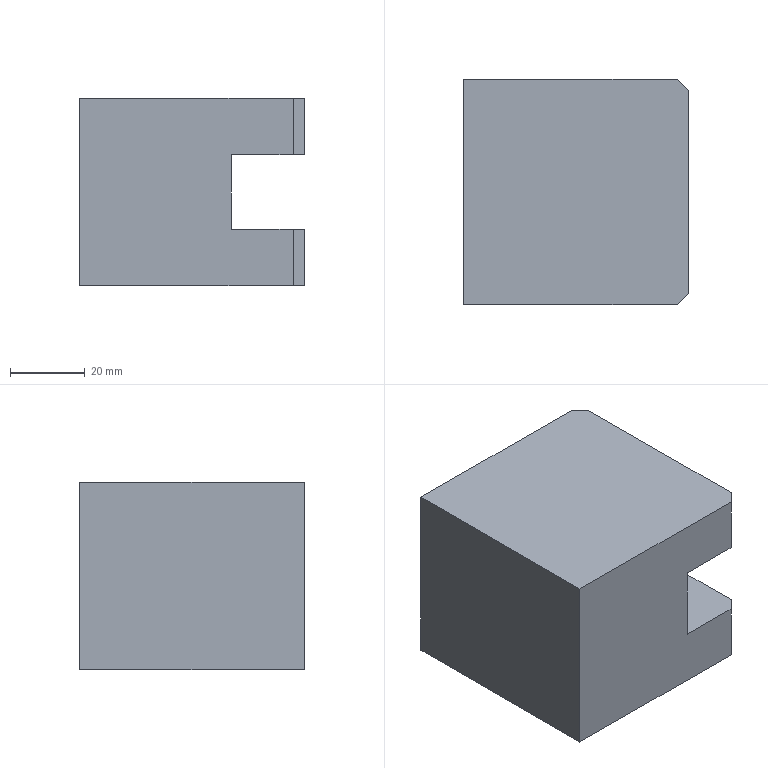Component | SolidWorks | Part52-1 | 1 solid | 14 faces | box 60 x 60 x 50 mm | volume 156330 mm3 | plane 14
build123d program:
from build123d import *

# Parameters (mm, degrees)
BOSS_EXTRUDE1_DEPTH = 30
CHAMFER1_SIZE       = 3


with BuildPart() as part:
    # Sketch1 → Boss-Extrude1 (new, symmetric)
    with BuildSketch(Plane(origin=(0, 0, 0), x_dir=(0, 0, -1), z_dir=(1, 0, 0))):
        Polygon((-25, 0), (25, 0), (25, 60), (10, 60), (10, 40.5), (-10, 40.5), (-10, 60), (-25, 60), align=None)
    extrude(amount=BOSS_EXTRUDE1_DEPTH, both=True)

    # Chamfer1
    chamfer1_edges = [part.edges().sort_by_distance(p)[0] for p in [
        (30, 60, -17.5),
        (30, 60, 17.5),
        (-30, 60, 17.5),
        (-30, 60, -17.5),
    ]]
    chamfer(chamfer1_edges, length=CHAMFER1_SIZE)


solid = part.part

# Placed as in the assembly
solid = solid.moved(Location((-265.007, 209, -385), (0, 0, -90)))
STEP:
#1=COLOUR_RGB('',0.7922,0.8196,0.9333);
#2=FILL_AREA_STYLE_COLOUR('',#1);
#3=FILL_AREA_STYLE('',(#2));
#4=SURFACE_STYLE_FILL_AREA(#3);
#5=SURFACE_SIDE_STYLE('',(#4));
#6=SURFACE_STYLE_USAGE(.BOTH.,#5);
#7=PRESENTATION_STYLE_ASSIGNMENT((#6));
#8=CARTESIAN_POINT('',(-8.071,7.165,-14.173));
#9=VERTEX_POINT('',#8);
#10=CARTESIAN_POINT('',(-8.071,9.291,-14.173));
#11=VERTEX_POINT('',#10);
#12=CARTESIAN_POINT('',(-8.071,7.047,-14.173));
#13=DIRECTION('',(0.,1.,0.));
#14=VECTOR('',#13,39.37);
#15=LINE('',#12,#14);
#16=EDGE_CURVE('',#9,#11,#15,.T.);
#17=ORIENTED_EDGE('',*,*,#16,.T.);
#18=CARTESIAN_POINT('',(-8.189,9.409,-14.173));
#19=VERTEX_POINT('',#18);
#20=CARTESIAN_POINT('',(-8.071,9.291,-14.173));
#21=DIRECTION('',(-0.7071,0.7071,0.));
#22=VECTOR('',#21,39.37);
#23=LINE('',#20,#22);
#24=EDGE_CURVE('',#11,#19,#23,.T.);
#25=ORIENTED_EDGE('',*,*,#24,.T.);
#26=CARTESIAN_POINT('',(-10.433,9.409,-14.173));
#27=VERTEX_POINT('',#26);
#28=CARTESIAN_POINT('',(-10.433,9.409,-14.173));
#29=DIRECTION('',(-1.,0.,0.));
#30=VECTOR('',#29,39.37);
#31=LINE('',#28,#30);
#32=EDGE_CURVE('',#19,#27,#31,.T.);
#33=ORIENTED_EDGE('',*,*,#32,.T.);
#34=CARTESIAN_POINT('',(-10.433,7.047,-14.173));
#35=VERTEX_POINT('',#34);
#36=CARTESIAN_POINT('',(-10.433,7.047,-14.173));
#37=DIRECTION('',(0.,1.,0.));
#38=VECTOR('',#37,39.37);
#39=LINE('',#36,#38);
#40=EDGE_CURVE('',#35,#27,#39,.T.);
#41=ORIENTED_EDGE('',*,*,#40,.F.);
#42=CARTESIAN_POINT('',(-8.189,7.047,-14.173));
#43=VERTEX_POINT('',#42);
#44=CARTESIAN_POINT('',(-10.433,7.047,-14.173));
#45=DIRECTION('',(-1.,0.,0.));
#46=VECTOR('',#45,39.37);
#47=LINE('',#44,#46);
#48=EDGE_CURVE('',#43,#35,#47,.T.);
#49=ORIENTED_EDGE('',*,*,#48,.F.);
#50=CARTESIAN_POINT('',(-8.189,7.047,-14.173));
#51=DIRECTION('',(0.7071,0.7071,0.));
#52=VECTOR('',#51,39.37);
#53=LINE('',#50,#52);
#54=EDGE_CURVE('',#43,#9,#53,.T.);
#55=ORIENTED_EDGE('',*,*,#54,.T.);
#56=EDGE_LOOP('',(#17,#25,#33,#41,#49,#55));
#57=FACE_OUTER_BOUND('',#56,.T.);
#58=CARTESIAN_POINT('',(-10.433,7.047,-14.173));
#59=DIRECTION('',(0.,0.,-1.));
#60=DIRECTION('',(0.,1.,0.));
#61=AXIS2_PLACEMENT_3D('',#58,#59,#60);
#62=PLANE('',#61);
#63=ADVANCED_FACE('',(#57),#62,.F.);
#64=CARTESIAN_POINT('',(-10.433,9.409,-16.142));
#65=VERTEX_POINT('',#64);
#66=CARTESIAN_POINT('',(-10.433,9.409,-14.173));
#67=DIRECTION('',(0.,0.,-1.));
#68=VECTOR('',#67,39.37);
#69=LINE('',#66,#68);
#70=EDGE_CURVE('',#27,#65,#69,.T.);
#71=ORIENTED_EDGE('',*,*,#70,.T.);
#72=CARTESIAN_POINT('',(-10.433,7.047,-16.142));
#73=VERTEX_POINT('',#72);
#74=CARTESIAN_POINT('',(-10.433,7.047,-16.142));
#75=DIRECTION('',(0.,1.,0.));
#76=VECTOR('',#75,39.37);
#77=LINE('',#74,#76);
#78=EDGE_CURVE('',#73,#65,#77,.T.);
#79=ORIENTED_EDGE('',*,*,#78,.F.);
#80=CARTESIAN_POINT('',(-10.433,7.047,-14.173));
#81=DIRECTION('',(0.,0.,-1.));
#82=VECTOR('',#81,39.37);
#83=LINE('',#80,#82);
#84=EDGE_CURVE('',#35,#73,#83,.T.);
#85=ORIENTED_EDGE('',*,*,#84,.F.);
#86=ORIENTED_EDGE('',*,*,#40,.T.);
#87=EDGE_LOOP('',(#71,#79,#85,#86));
#88=FACE_OUTER_BOUND('',#87,.T.);
#89=CARTESIAN_POINT('',(-10.433,7.047,-14.173));
#90=DIRECTION('',(1.,0.,0.));
#91=DIRECTION('',(0.,0.,1.));
#92=AXIS2_PLACEMENT_3D('',#89,#90,#91);
#93=PLANE('',#92);
#94=ADVANCED_FACE('',(#88),#93,.F.);
#95=CARTESIAN_POINT('',(-8.189,9.409,-16.142));
#96=VERTEX_POINT('',#95);
#97=CARTESIAN_POINT('',(-10.433,9.409,-16.142));
#98=DIRECTION('',(1.,0.,0.));
#99=VECTOR('',#98,39.37);
#100=LINE('',#97,#99);
#101=EDGE_CURVE('',#65,#96,#100,.T.);
#102=ORIENTED_EDGE('',*,*,#101,.T.);
#103=CARTESIAN_POINT('',(-8.071,9.291,-16.142));
#104=VERTEX_POINT('',#103);
#105=CARTESIAN_POINT('',(-8.071,9.291,-16.142));
#106=DIRECTION('',(0.7071,-0.7071,0.));
#107=VECTOR('',#106,39.37);
#108=LINE('',#105,#107);
#109=EDGE_CURVE('',#96,#104,#108,.T.);
#110=ORIENTED_EDGE('',*,*,#109,.T.);
#111=CARTESIAN_POINT('',(-8.071,7.165,-16.142));
#112=VERTEX_POINT('',#111);
#113=CARTESIAN_POINT('',(-8.071,7.047,-16.142));
#114=DIRECTION('',(0.,1.,0.));
#115=VECTOR('',#114,39.37);
#116=LINE('',#113,#115);
#117=EDGE_CURVE('',#112,#104,#116,.T.);
#118=ORIENTED_EDGE('',*,*,#117,.F.);
#119=CARTESIAN_POINT('',(-8.189,7.047,-16.142));
#120=VERTEX_POINT('',#119);
#121=CARTESIAN_POINT('',(-8.189,7.047,-16.142));
#122=DIRECTION('',(-0.7071,-0.7071,0.));
#123=VECTOR('',#122,39.37);
#124=LINE('',#121,#123);
#125=EDGE_CURVE('',#112,#120,#124,.T.);
#126=ORIENTED_EDGE('',*,*,#125,.T.);
#127=CARTESIAN_POINT('',(-10.433,7.047,-16.142));
#128=DIRECTION('',(1.,0.,0.));
#129=VECTOR('',#128,39.37);
#130=LINE('',#127,#129);
#131=EDGE_CURVE('',#73,#120,#130,.T.);
#132=ORIENTED_EDGE('',*,*,#131,.F.);
#133=ORIENTED_EDGE('',*,*,#78,.T.);
#134=EDGE_LOOP('',(#102,#110,#118,#126,#132,#133));
#135=FACE_OUTER_BOUND('',#134,.T.);
#136=CARTESIAN_POINT('',(-10.433,7.047,-16.142));
#137=DIRECTION('',(0.,0.,1.));
#138=DIRECTION('',(0.,-1.,0.));
#139=AXIS2_PLACEMENT_3D('',#136,#137,#138);
#140=PLANE('',#139);
#141=ADVANCED_FACE('',(#135),#140,.F.);
#142=ORIENTED_EDGE('',*,*,#117,.T.);
#143=CARTESIAN_POINT('',(-8.071,9.291,-15.551));
#144=VERTEX_POINT('',#143);
#145=CARTESIAN_POINT('',(-8.071,9.291,-15.551));
#146=DIRECTION('',(0.,0.,1.));
#147=VECTOR('',#146,39.37);
#148=LINE('',#145,#147);
#149=EDGE_CURVE('',#104,#144,#148,.T.);
#150=ORIENTED_EDGE('',*,*,#149,.T.);
#151=CARTESIAN_POINT('',(-8.071,7.165,-15.551));
#152=VERTEX_POINT('',#151);
#153=CARTESIAN_POINT('',(-8.071,7.047,-15.551));
#154=DIRECTION('',(0.,1.,0.));
#155=VECTOR('',#154,39.37);
#156=LINE('',#153,#155);
#157=EDGE_CURVE('',#152,#144,#156,.T.);
#158=ORIENTED_EDGE('',*,*,#157,.F.);
#159=CARTESIAN_POINT('',(-8.071,7.165,-15.551));
#160=DIRECTION('',(0.,0.,-1.));
#161=VECTOR('',#160,39.37);
#162=LINE('',#159,#161);
#163=EDGE_CURVE('',#152,#112,#162,.T.);
#164=ORIENTED_EDGE('',*,*,#163,.T.);
#165=EDGE_LOOP('',(#142,#150,#158,#164));
#166=FACE_OUTER_BOUND('',#165,.T.);
#167=CARTESIAN_POINT('',(-8.071,7.047,-15.551));
#168=DIRECTION('',(-1.,0.,0.));
#169=DIRECTION('',(0.,0.,-1.));
#170=AXIS2_PLACEMENT_3D('',#167,#168,#169);
#171=PLANE('',#170);
#172=ADVANCED_FACE('',(#166),#171,.F.);
#173=ORIENTED_EDGE('',*,*,#157,.T.);
#174=CARTESIAN_POINT('',(-8.189,9.409,-15.551));
#175=VERTEX_POINT('',#174);
#176=CARTESIAN_POINT('',(-8.071,9.291,-15.551));
#177=DIRECTION('',(-0.7071,0.7071,-0.));
#178=VECTOR('',#177,39.37);
#179=LINE('',#176,#178);
#180=EDGE_CURVE('',#144,#175,#179,.T.);
#181=ORIENTED_EDGE('',*,*,#180,.T.);
#182=CARTESIAN_POINT('',(-8.839,9.409,-15.551));
#183=VERTEX_POINT('',#182);
#184=CARTESIAN_POINT('',(-8.071,9.409,-15.551));
#185=DIRECTION('',(-1.,0.,-0.));
#186=VECTOR('',#185,39.37);
#187=LINE('',#184,#186);
#188=EDGE_CURVE('',#175,#183,#187,.T.);
#189=ORIENTED_EDGE('',*,*,#188,.T.);
#190=CARTESIAN_POINT('',(-8.839,7.047,-15.551));
#191=VERTEX_POINT('',#190);
#192=CARTESIAN_POINT('',(-8.839,7.047,-15.551));
#193=DIRECTION('',(0.,1.,0.));
#194=VECTOR('',#193,39.37);
#195=LINE('',#192,#194);
#196=EDGE_CURVE('',#191,#183,#195,.T.);
#197=ORIENTED_EDGE('',*,*,#196,.F.);
#198=CARTESIAN_POINT('',(-8.189,7.047,-15.551));
#199=VERTEX_POINT('',#198);
#200=CARTESIAN_POINT('',(-8.071,7.047,-15.551));
#201=DIRECTION('',(-1.,0.,-0.));
#202=VECTOR('',#201,39.37);
#203=LINE('',#200,#202);
#204=EDGE_CURVE('',#199,#191,#203,.T.);
#205=ORIENTED_EDGE('',*,*,#204,.F.);
#206=CARTESIAN_POINT('',(-8.189,7.047,-15.551));
#207=DIRECTION('',(0.7071,0.7071,0.));
#208=VECTOR('',#207,39.37);
#209=LINE('',#206,#208);
#210=EDGE_CURVE('',#199,#152,#209,.T.);
#211=ORIENTED_EDGE('',*,*,#210,.T.);
#212=EDGE_LOOP('',(#173,#181,#189,#197,#205,#211));
#213=FACE_OUTER_BOUND('',#212,.T.);
#214=CARTESIAN_POINT('',(-8.071,7.047,-15.551));
#215=DIRECTION('',(0.,0.,-1.));
#216=DIRECTION('',(1.,0.,0.));
#217=AXIS2_PLACEMENT_3D('',#214,#215,#216);
#218=PLANE('',#217);
#219=ADVANCED_FACE('',(#213),#218,.F.);
#220=CARTESIAN_POINT('',(-8.839,9.409,-14.764));
#221=VERTEX_POINT('',#220);
#222=CARTESIAN_POINT('',(-8.839,9.409,-14.764));
#223=DIRECTION('',(0.,0.,1.));
#224=VECTOR('',#223,39.37);
#225=LINE('',#222,#224);
#226=EDGE_CURVE('',#183,#221,#225,.T.);
#227=ORIENTED_EDGE('',*,*,#226,.T.);
#228=CARTESIAN_POINT('',(-8.839,7.047,-14.764));
#229=VERTEX_POINT('',#228);
#230=CARTESIAN_POINT('',(-8.839,7.047,-14.764));
#231=DIRECTION('',(0.,1.,0.));
#232=VECTOR('',#231,39.37);
#233=LINE('',#230,#232);
#234=EDGE_CURVE('',#229,#221,#233,.T.);
#235=ORIENTED_EDGE('',*,*,#234,.F.);
#236=CARTESIAN_POINT('',(-8.839,7.047,-14.764));
#237=DIRECTION('',(0.,0.,1.));
#238=VECTOR('',#237,39.37);
#239=LINE('',#236,#238);
#240=EDGE_CURVE('',#191,#229,#239,.T.);
#241=ORIENTED_EDGE('',*,*,#240,.F.);
#242=ORIENTED_EDGE('',*,*,#196,.T.);
#243=EDGE_LOOP('',(#227,#235,#241,#242));
#244=FACE_OUTER_BOUND('',#243,.T.);
#245=CARTESIAN_POINT('',(-8.839,7.047,-14.764));
#246=DIRECTION('',(-1.,0.,0.));
#247=DIRECTION('',(0.,0.,-1.));
#248=AXIS2_PLACEMENT_3D('',#245,#246,#247);
#249=PLANE('',#248);
#250=ADVANCED_FACE('',(#244),#249,.F.);
#251=CARTESIAN_POINT('',(-8.189,9.409,-14.764));
#252=VERTEX_POINT('',#251);
#253=CARTESIAN_POINT('',(-8.071,9.409,-14.764));
#254=DIRECTION('',(1.,0.,0.));
#255=VECTOR('',#254,39.37);
#256=LINE('',#253,#255);
#257=EDGE_CURVE('',#221,#252,#256,.T.);
#258=ORIENTED_EDGE('',*,*,#257,.T.);
#259=CARTESIAN_POINT('',(-8.071,9.291,-14.764));
#260=VERTEX_POINT('',#259);
#261=CARTESIAN_POINT('',(-8.071,9.291,-14.764));
#262=DIRECTION('',(0.7071,-0.7071,0.));
#263=VECTOR('',#262,39.37);
#264=LINE('',#261,#263);
#265=EDGE_CURVE('',#252,#260,#264,.T.);
#266=ORIENTED_EDGE('',*,*,#265,.T.);
#267=CARTESIAN_POINT('',(-8.071,7.165,-14.764));
#268=VERTEX_POINT('',#267);
#269=CARTESIAN_POINT('',(-8.071,7.047,-14.764));
#270=DIRECTION('',(0.,1.,0.));
#271=VECTOR('',#270,39.37);
#272=LINE('',#269,#271);
#273=EDGE_CURVE('',#268,#260,#272,.T.);
#274=ORIENTED_EDGE('',*,*,#273,.F.);
#275=CARTESIAN_POINT('',(-8.189,7.047,-14.764));
#276=VERTEX_POINT('',#275);
#277=CARTESIAN_POINT('',(-8.189,7.047,-14.764));
#278=DIRECTION('',(-0.7071,-0.7071,-0.));
#279=VECTOR('',#278,39.37);
#280=LINE('',#277,#279);
#281=EDGE_CURVE('',#268,#276,#280,.T.);
#282=ORIENTED_EDGE('',*,*,#281,.T.);
#283=CARTESIAN_POINT('',(-8.071,7.047,-14.764));
#284=DIRECTION('',(1.,0.,0.));
#285=VECTOR('',#284,39.37);
#286=LINE('',#283,#285);
#287=EDGE_CURVE('',#229,#276,#286,.T.);
#288=ORIENTED_EDGE('',*,*,#287,.F.);
#289=ORIENTED_EDGE('',*,*,#234,.T.);
#290=EDGE_LOOP('',(#258,#266,#274,#282,#288,#289));
#291=FACE_OUTER_BOUND('',#290,.T.);
#292=CARTESIAN_POINT('',(-8.071,7.047,-14.764));
#293=DIRECTION('',(-0.,0.,1.));
#294=DIRECTION('',(-1.,0.,-0.));
#295=AXIS2_PLACEMENT_3D('',#292,#293,#294);
#296=PLANE('',#295);
#297=ADVANCED_FACE('',(#291),#296,.F.);
#298=ORIENTED_EDGE('',*,*,#273,.T.);
#299=CARTESIAN_POINT('',(-8.071,9.291,-14.173));
#300=DIRECTION('',(0.,0.,1.));
#301=VECTOR('',#300,39.37);
#302=LINE('',#299,#301);
#303=EDGE_CURVE('',#260,#11,#302,.T.);
#304=ORIENTED_EDGE('',*,*,#303,.T.);
#305=ORIENTED_EDGE('',*,*,#16,.F.);
#306=CARTESIAN_POINT('',(-8.071,7.165,-14.173));
#307=DIRECTION('',(0.,0.,-1.));
#308=VECTOR('',#307,39.37);
#309=LINE('',#306,#308);
#310=EDGE_CURVE('',#9,#268,#309,.T.);
#311=ORIENTED_EDGE('',*,*,#310,.T.);
#312=EDGE_LOOP('',(#298,#304,#305,#311));
#313=FACE_OUTER_BOUND('',#312,.T.);
#314=CARTESIAN_POINT('',(-8.071,7.047,-14.173));
#315=DIRECTION('',(-1.,0.,0.));
#316=DIRECTION('',(0.,0.,-1.));
#317=AXIS2_PLACEMENT_3D('',#314,#315,#316);
#318=PLANE('',#317);
#319=ADVANCED_FACE('',(#313),#318,.F.);
#320=ORIENTED_EDGE('',*,*,#287,.T.);
#321=CARTESIAN_POINT('',(-8.189,7.047,-15.157));
#322=DIRECTION('',(0.,0.,1.));
#323=VECTOR('',#322,39.37);
#324=LINE('',#321,#323);
#325=EDGE_CURVE('',#276,#43,#324,.T.);
#326=ORIENTED_EDGE('',*,*,#325,.T.);
#327=ORIENTED_EDGE('',*,*,#48,.T.);
#328=ORIENTED_EDGE('',*,*,#84,.T.);
#329=ORIENTED_EDGE('',*,*,#131,.T.);
#330=CARTESIAN_POINT('',(-8.189,7.047,-15.157));
#331=DIRECTION('',(0.,0.,1.));
#332=VECTOR('',#331,39.37);
#333=LINE('',#330,#332);
#334=EDGE_CURVE('',#120,#199,#333,.T.);
#335=ORIENTED_EDGE('',*,*,#334,.T.);
#336=ORIENTED_EDGE('',*,*,#204,.T.);
#337=ORIENTED_EDGE('',*,*,#240,.T.);
#338=EDGE_LOOP('',(#320,#326,#327,#328,#329,#335,#336,#337));
#339=FACE_OUTER_BOUND('',#338,.T.);
#340=CARTESIAN_POINT('',(-10.433,7.047,-15.157));
#341=DIRECTION('',(0.,1.,0.));
#342=DIRECTION('',(0.,0.,1.));
#343=AXIS2_PLACEMENT_3D('',#340,#341,#342);
#344=PLANE('',#343);
#345=ADVANCED_FACE('',(#339),#344,.F.);
#346=ORIENTED_EDGE('',*,*,#32,.F.);
#347=CARTESIAN_POINT('',(-8.189,9.409,-14.764));
#348=DIRECTION('',(0.,0.,-1.));
#349=VECTOR('',#348,39.37);
#350=LINE('',#347,#349);
#351=EDGE_CURVE('',#19,#252,#350,.T.);
#352=ORIENTED_EDGE('',*,*,#351,.T.);
#353=ORIENTED_EDGE('',*,*,#257,.F.);
#354=ORIENTED_EDGE('',*,*,#226,.F.);
#355=ORIENTED_EDGE('',*,*,#188,.F.);
#356=CARTESIAN_POINT('',(-8.189,9.409,-16.142));
#357=DIRECTION('',(0.,0.,-1.));
#358=VECTOR('',#357,39.37);
#359=LINE('',#356,#358);
#360=EDGE_CURVE('',#175,#96,#359,.T.);
#361=ORIENTED_EDGE('',*,*,#360,.T.);
#362=ORIENTED_EDGE('',*,*,#101,.F.);
#363=ORIENTED_EDGE('',*,*,#70,.F.);
#364=EDGE_LOOP('',(#346,#352,#353,#354,#355,#361,#362,#363));
#365=FACE_OUTER_BOUND('',#364,.T.);
#366=CARTESIAN_POINT('',(-10.433,9.409,-15.157));
#367=DIRECTION('',(0.,1.,0.));
#368=DIRECTION('',(0.,0.,1.));
#369=AXIS2_PLACEMENT_3D('',#366,#367,#368);
#370=PLANE('',#369);
#371=ADVANCED_FACE('',(#365),#370,.T.);
#372=ORIENTED_EDGE('',*,*,#265,.F.);
#373=ORIENTED_EDGE('',*,*,#351,.F.);
#374=ORIENTED_EDGE('',*,*,#24,.F.);
#375=ORIENTED_EDGE('',*,*,#303,.F.);
#376=EDGE_LOOP('',(#372,#373,#374,#375));
#377=FACE_OUTER_BOUND('',#376,.T.);
#378=CARTESIAN_POINT('',(-8.071,9.291,-14.173));
#379=DIRECTION('',(0.7071,0.7071,0.));
#380=DIRECTION('',(0.,0.,-1.));
#381=AXIS2_PLACEMENT_3D('',#378,#379,#380);
#382=PLANE('',#381);
#383=ADVANCED_FACE('',(#377),#382,.T.);
#384=ORIENTED_EDGE('',*,*,#109,.F.);
#385=ORIENTED_EDGE('',*,*,#360,.F.);
#386=ORIENTED_EDGE('',*,*,#180,.F.);
#387=ORIENTED_EDGE('',*,*,#149,.F.);
#388=EDGE_LOOP('',(#384,#385,#386,#387));
#389=FACE_OUTER_BOUND('',#388,.T.);
#390=CARTESIAN_POINT('',(-8.071,9.291,-15.551));
#391=DIRECTION('',(0.7071,0.7071,0.));
#392=DIRECTION('',(0.,0.,-1.));
#393=AXIS2_PLACEMENT_3D('',#390,#391,#392);
#394=PLANE('',#393);
#395=ADVANCED_FACE('',(#389),#394,.T.);
#396=ORIENTED_EDGE('',*,*,#281,.F.);
#397=ORIENTED_EDGE('',*,*,#310,.F.);
#398=ORIENTED_EDGE('',*,*,#54,.F.);
#399=ORIENTED_EDGE('',*,*,#325,.F.);
#400=EDGE_LOOP('',(#396,#397,#398,#399));
#401=FACE_OUTER_BOUND('',#400,.T.);
#402=CARTESIAN_POINT('',(-8.189,7.047,-15.157));
#403=DIRECTION('',(-0.7071,0.7071,0.));
#404=DIRECTION('',(0.,0.,1.));
#405=AXIS2_PLACEMENT_3D('',#402,#403,#404);
#406=PLANE('',#405);
#407=ADVANCED_FACE('',(#401),#406,.F.);
#408=ORIENTED_EDGE('',*,*,#125,.F.);
#409=ORIENTED_EDGE('',*,*,#163,.F.);
#410=ORIENTED_EDGE('',*,*,#210,.F.);
#411=ORIENTED_EDGE('',*,*,#334,.F.);
#412=EDGE_LOOP('',(#408,#409,#410,#411));
#413=FACE_OUTER_BOUND('',#412,.T.);
#414=CARTESIAN_POINT('',(-8.189,7.047,-15.157));
#415=DIRECTION('',(-0.7071,0.7071,0.));
#416=DIRECTION('',(0.,0.,1.));
#417=AXIS2_PLACEMENT_3D('',#414,#415,#416);
#418=PLANE('',#417);
#419=ADVANCED_FACE('',(#413),#418,.F.);
#420=CLOSED_SHELL('',(#63,#94,#141,#172,#219,#250,#297,#319,#345,#371,#383,#395,#407,#419));
#421=MANIFOLD_SOLID_BREP('',#420);
#422=STYLED_ITEM('',(#7),#421);
#423=PRESENTATION_LAYER_ASSIGNMENT('','',(#422));
#424=CARTESIAN_POINT('',(0.,0.,0.));
#425=DIRECTION('',(0.,0.,1.));
#426=DIRECTION('',(1.,0.,0.));
#427=AXIS2_PLACEMENT_3D('',#424,#425,#426);
#428=(LENGTH_UNIT()NAMED_UNIT(*)SI_UNIT($,.METRE.));
#429=LENGTH_MEASURE_WITH_UNIT(LENGTH_MEASURE(0.0254),#428);
#430=DIMENSIONAL_EXPONENTS(1.,0.,0.,0.,0.,0.,0.);
#431=(CONVERSION_BASED_UNIT('',#429)LENGTH_UNIT()NAMED_UNIT(#430));
#432=UNCERTAINTY_MEASURE_WITH_UNIT(LENGTH_MEASURE(0.00001),#431,'','');
#433=(NAMED_UNIT(*)PLANE_ANGLE_UNIT()SI_UNIT($,.RADIAN.));
#434=(NAMED_UNIT(*)SI_UNIT($,.STERADIAN.)SOLID_ANGLE_UNIT());
#435=(GEOMETRIC_REPRESENTATION_CONTEXT(3)GLOBAL_UNCERTAINTY_ASSIGNED_CONTEXT((#432))GLOBAL_UNIT_ASSIGNED_CONTEXT((#431,#433,#434))REPRESENTATION_CONTEXT('',''));
#436=ADVANCED_BREP_SHAPE_REPRESENTATION('',(#421,#427),#435);
#437=(LENGTH_UNIT()NAMED_UNIT(*)SI_UNIT($,.METRE.));
#438=LENGTH_MEASURE_WITH_UNIT(LENGTH_MEASURE(0.0254),#437);
#439=DIMENSIONAL_EXPONENTS(1.,0.,0.,0.,0.,0.,0.);
#440=(CONVERSION_BASED_UNIT('',#438)LENGTH_UNIT()NAMED_UNIT(#439));
#441=UNCERTAINTY_MEASURE_WITH_UNIT(LENGTH_MEASURE(0.00001),#440,'','');
#442=(NAMED_UNIT(*)PLANE_ANGLE_UNIT()SI_UNIT($,.RADIAN.));
#443=(NAMED_UNIT(*)SI_UNIT($,.STERADIAN.)SOLID_ANGLE_UNIT());
#444=(GEOMETRIC_REPRESENTATION_CONTEXT(3)GLOBAL_UNCERTAINTY_ASSIGNED_CONTEXT((#441))GLOBAL_UNIT_ASSIGNED_CONTEXT((#440,#442,#443))REPRESENTATION_CONTEXT('',''));
#445=MECHANICAL_DESIGN_GEOMETRIC_PRESENTATION_REPRESENTATION('',(#422),#444);